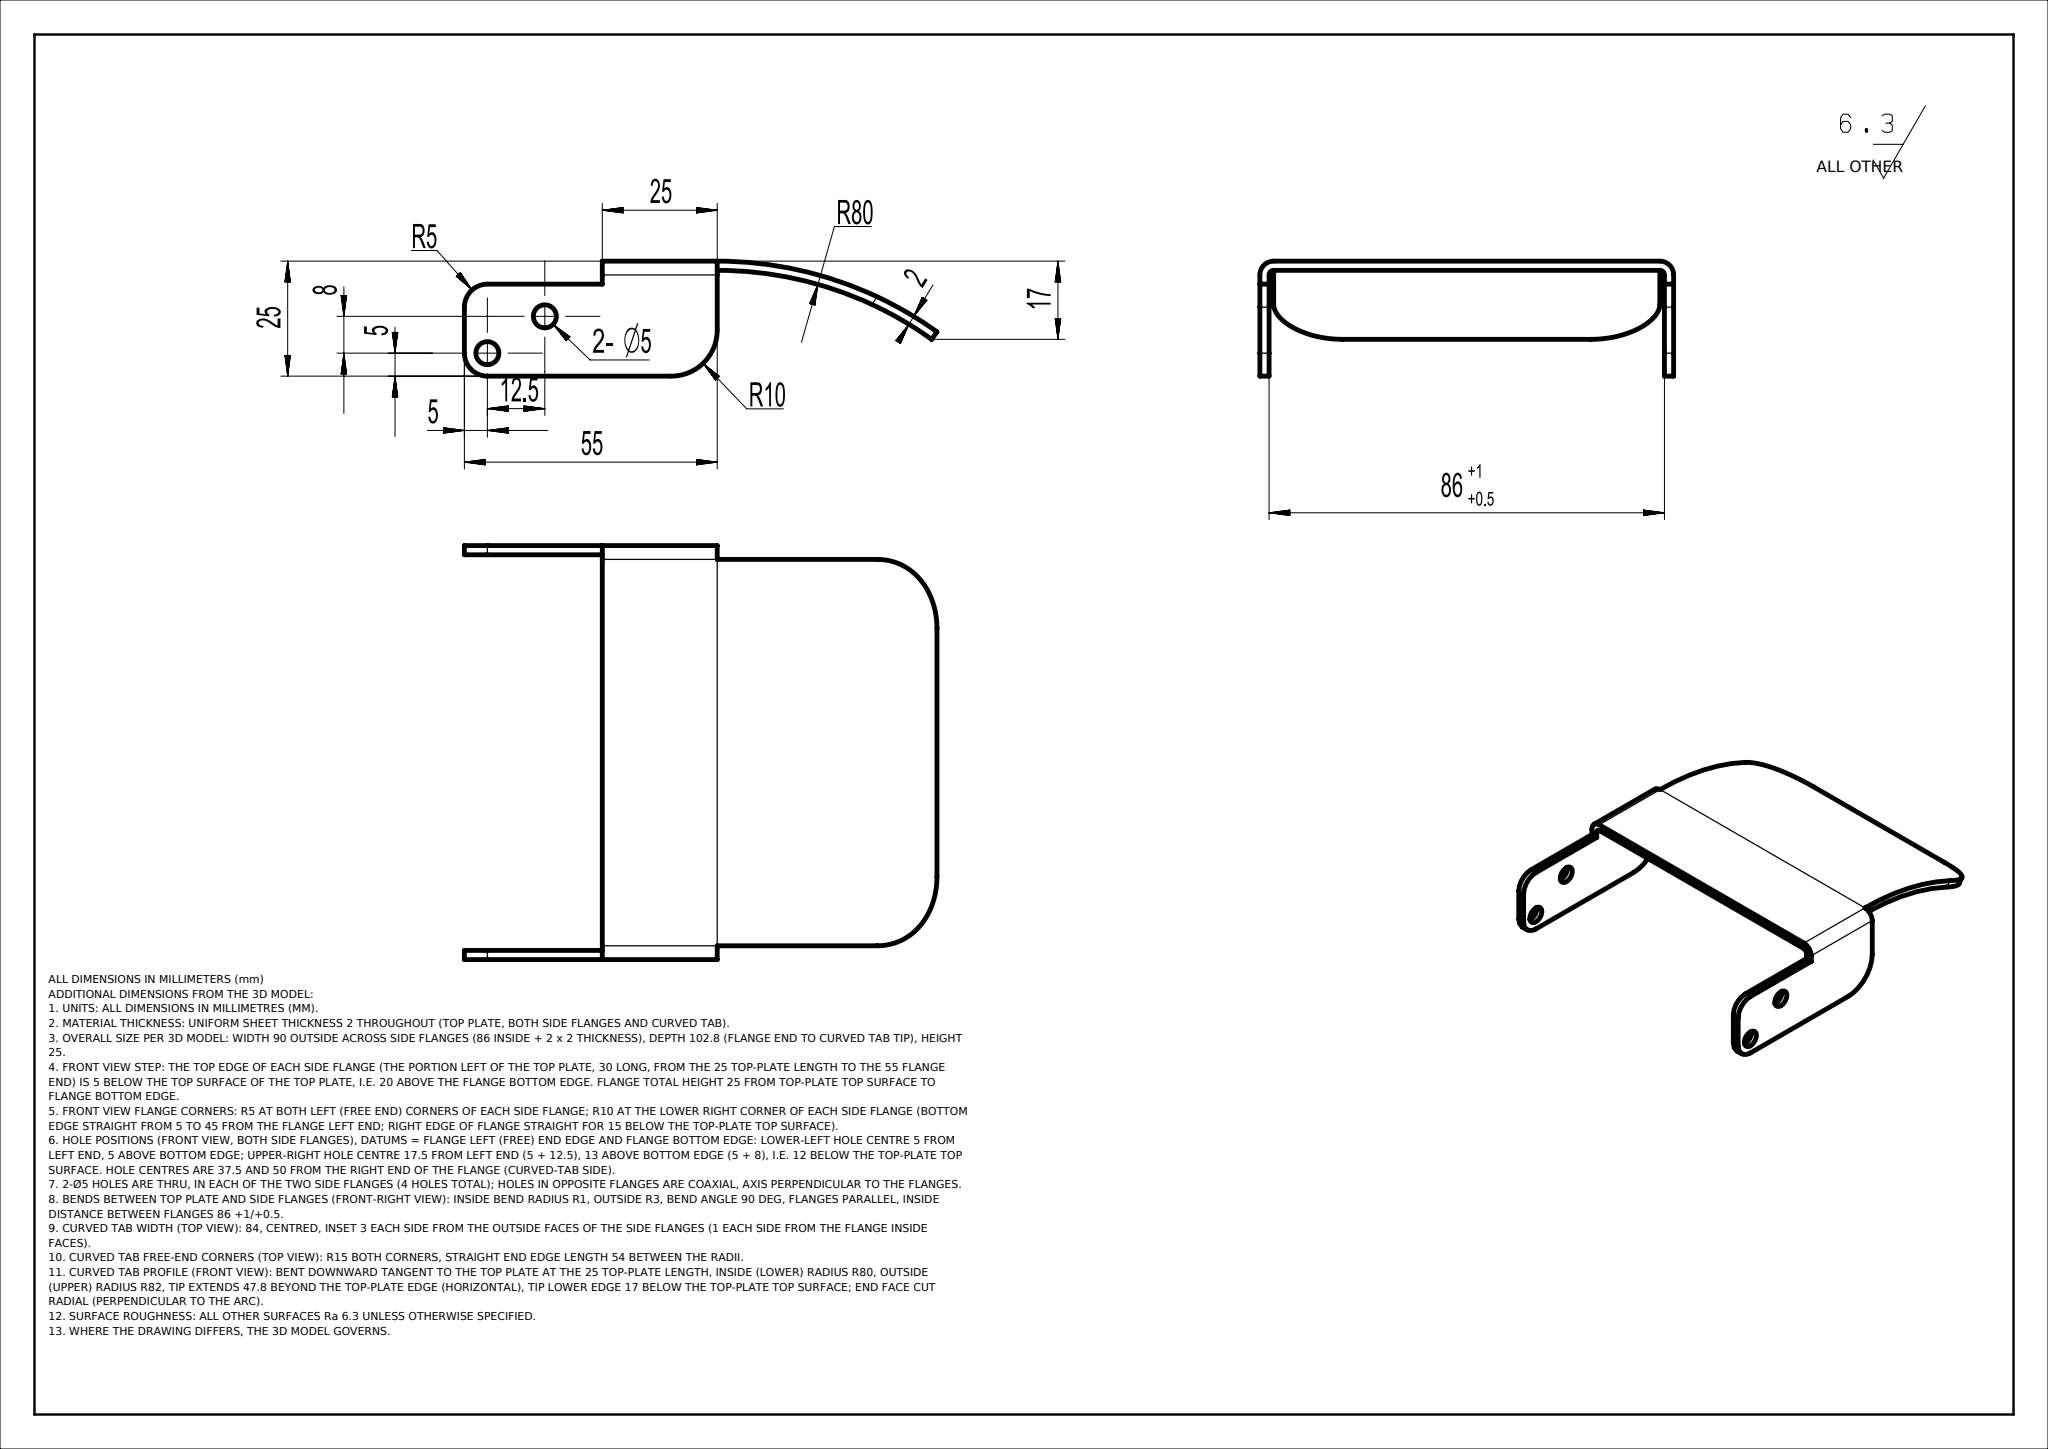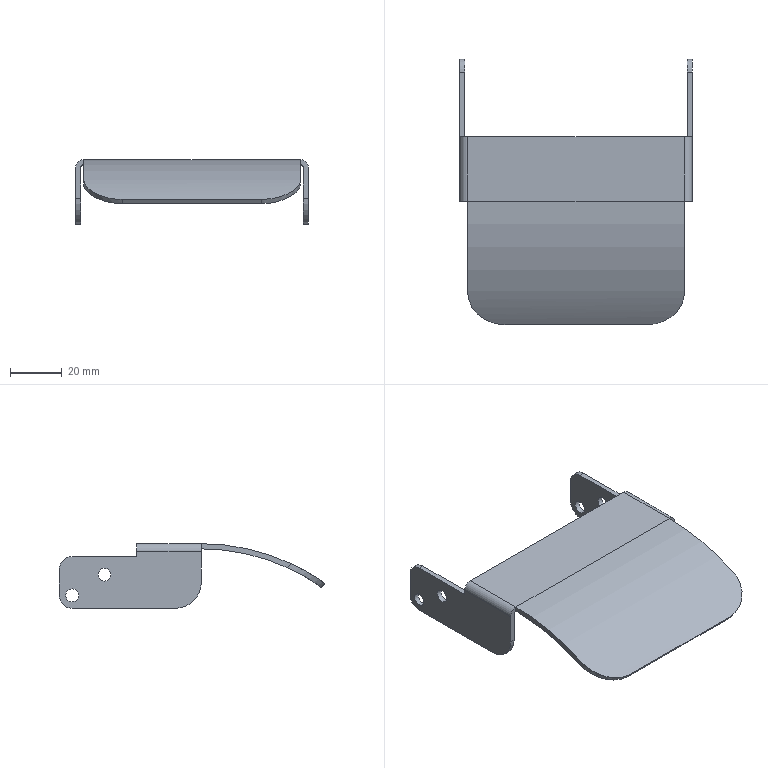Part | NX | mm | 1 solid | 36 faces | box 90 x 102.8 x 25 mm | volume 17104 mm3 | plane 18 | cylinder 18 | commonest cylinder face diameters 10 x4 5 x4 2 x2 6 x2 30 x2 20 x2 160 x1 164 x1